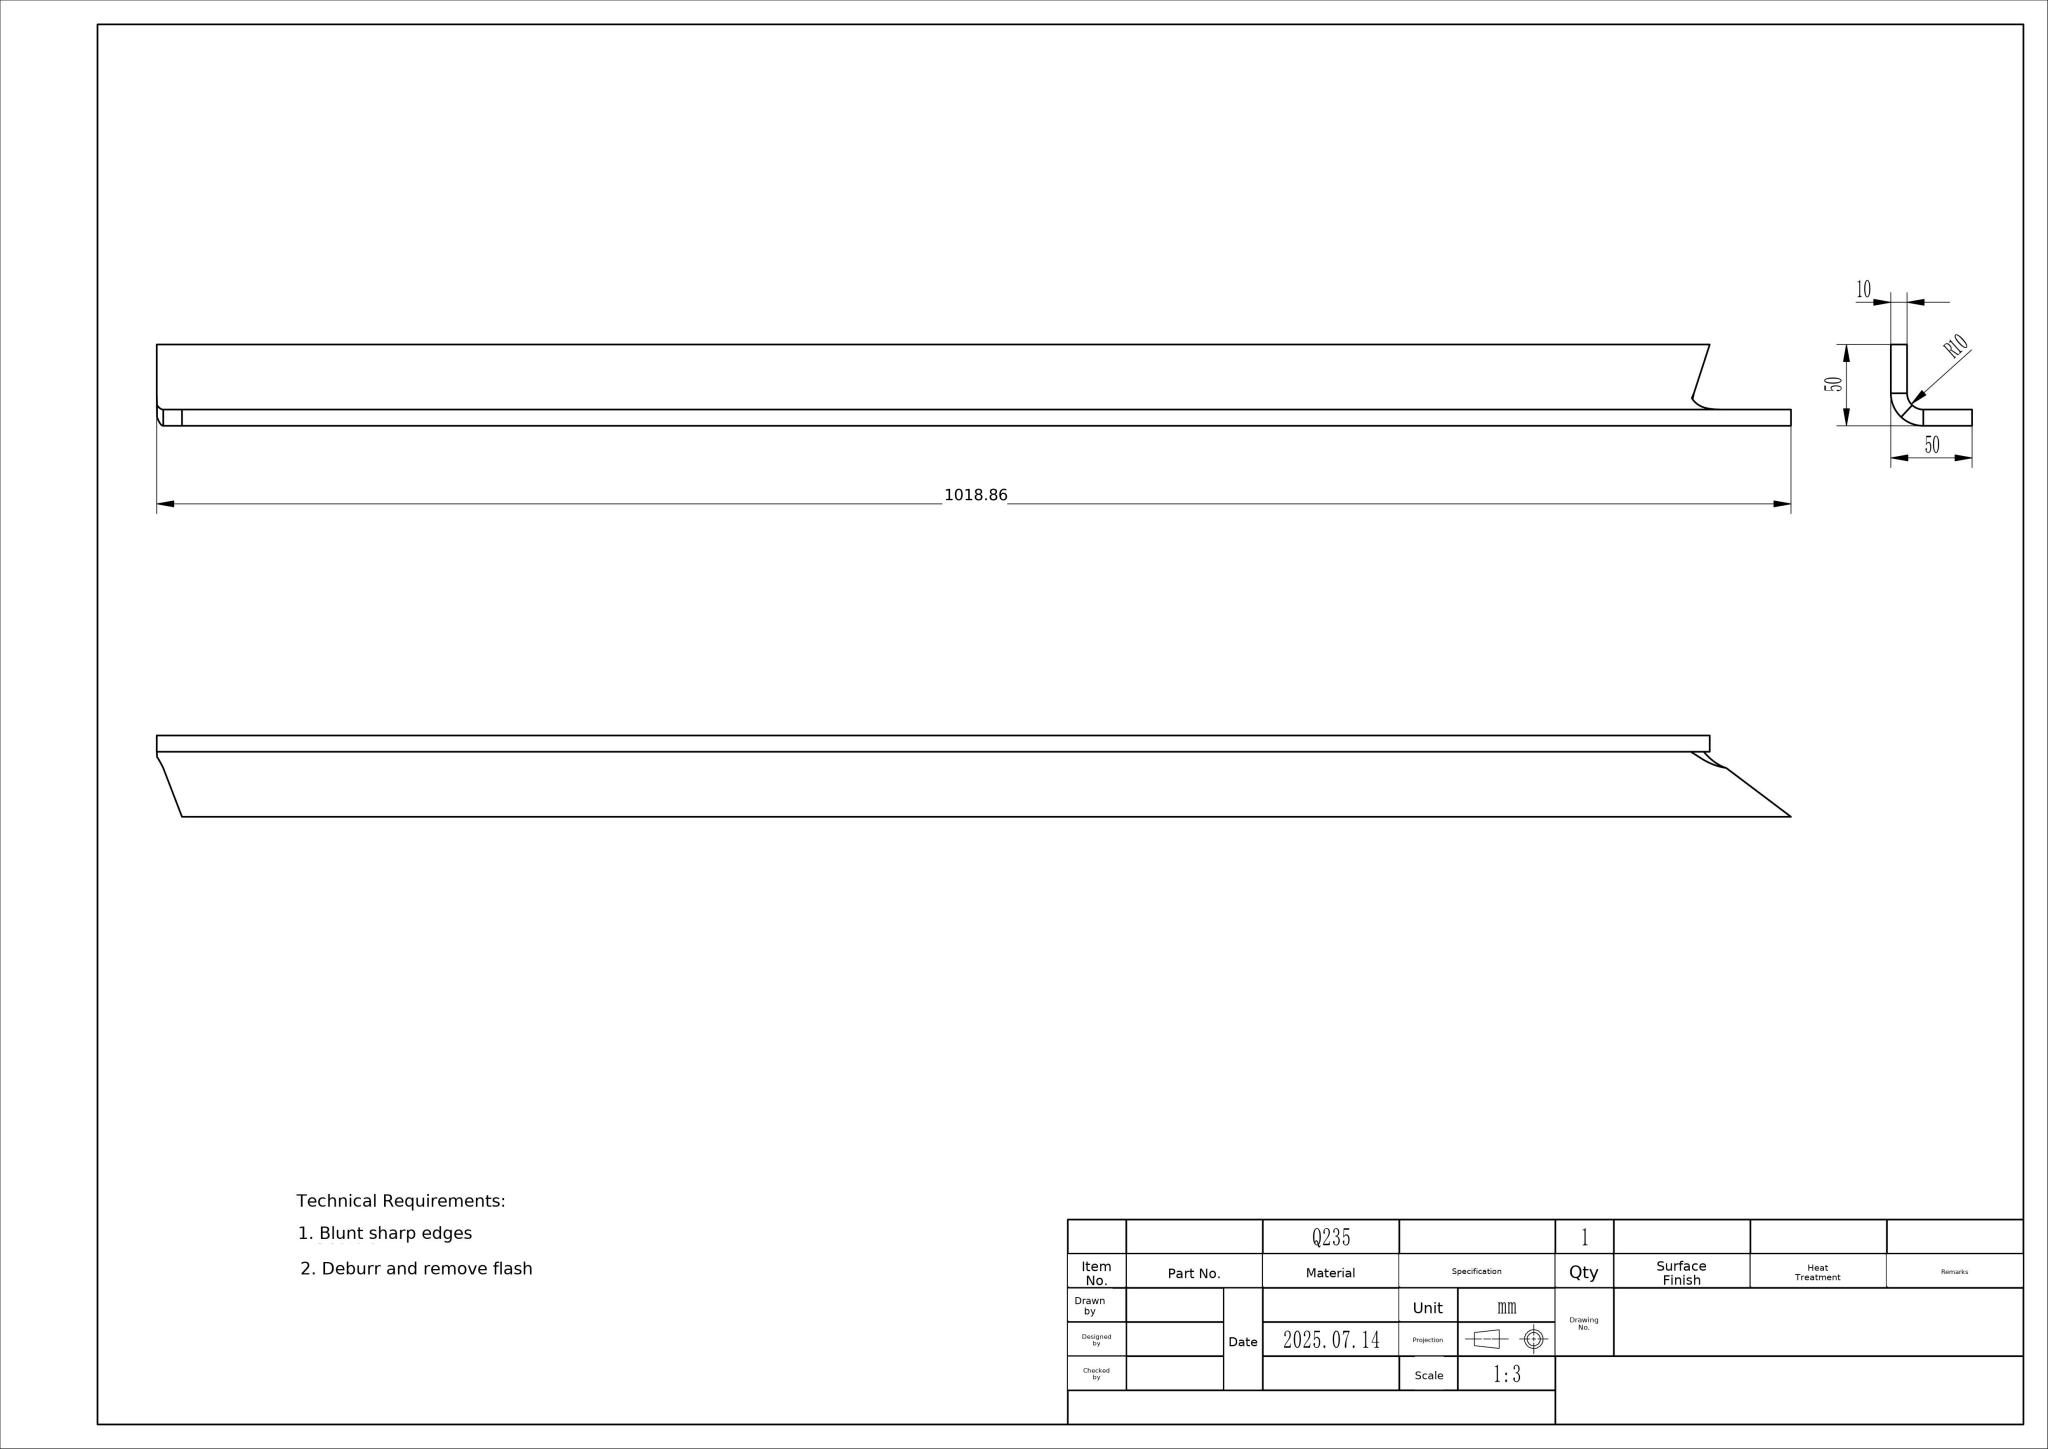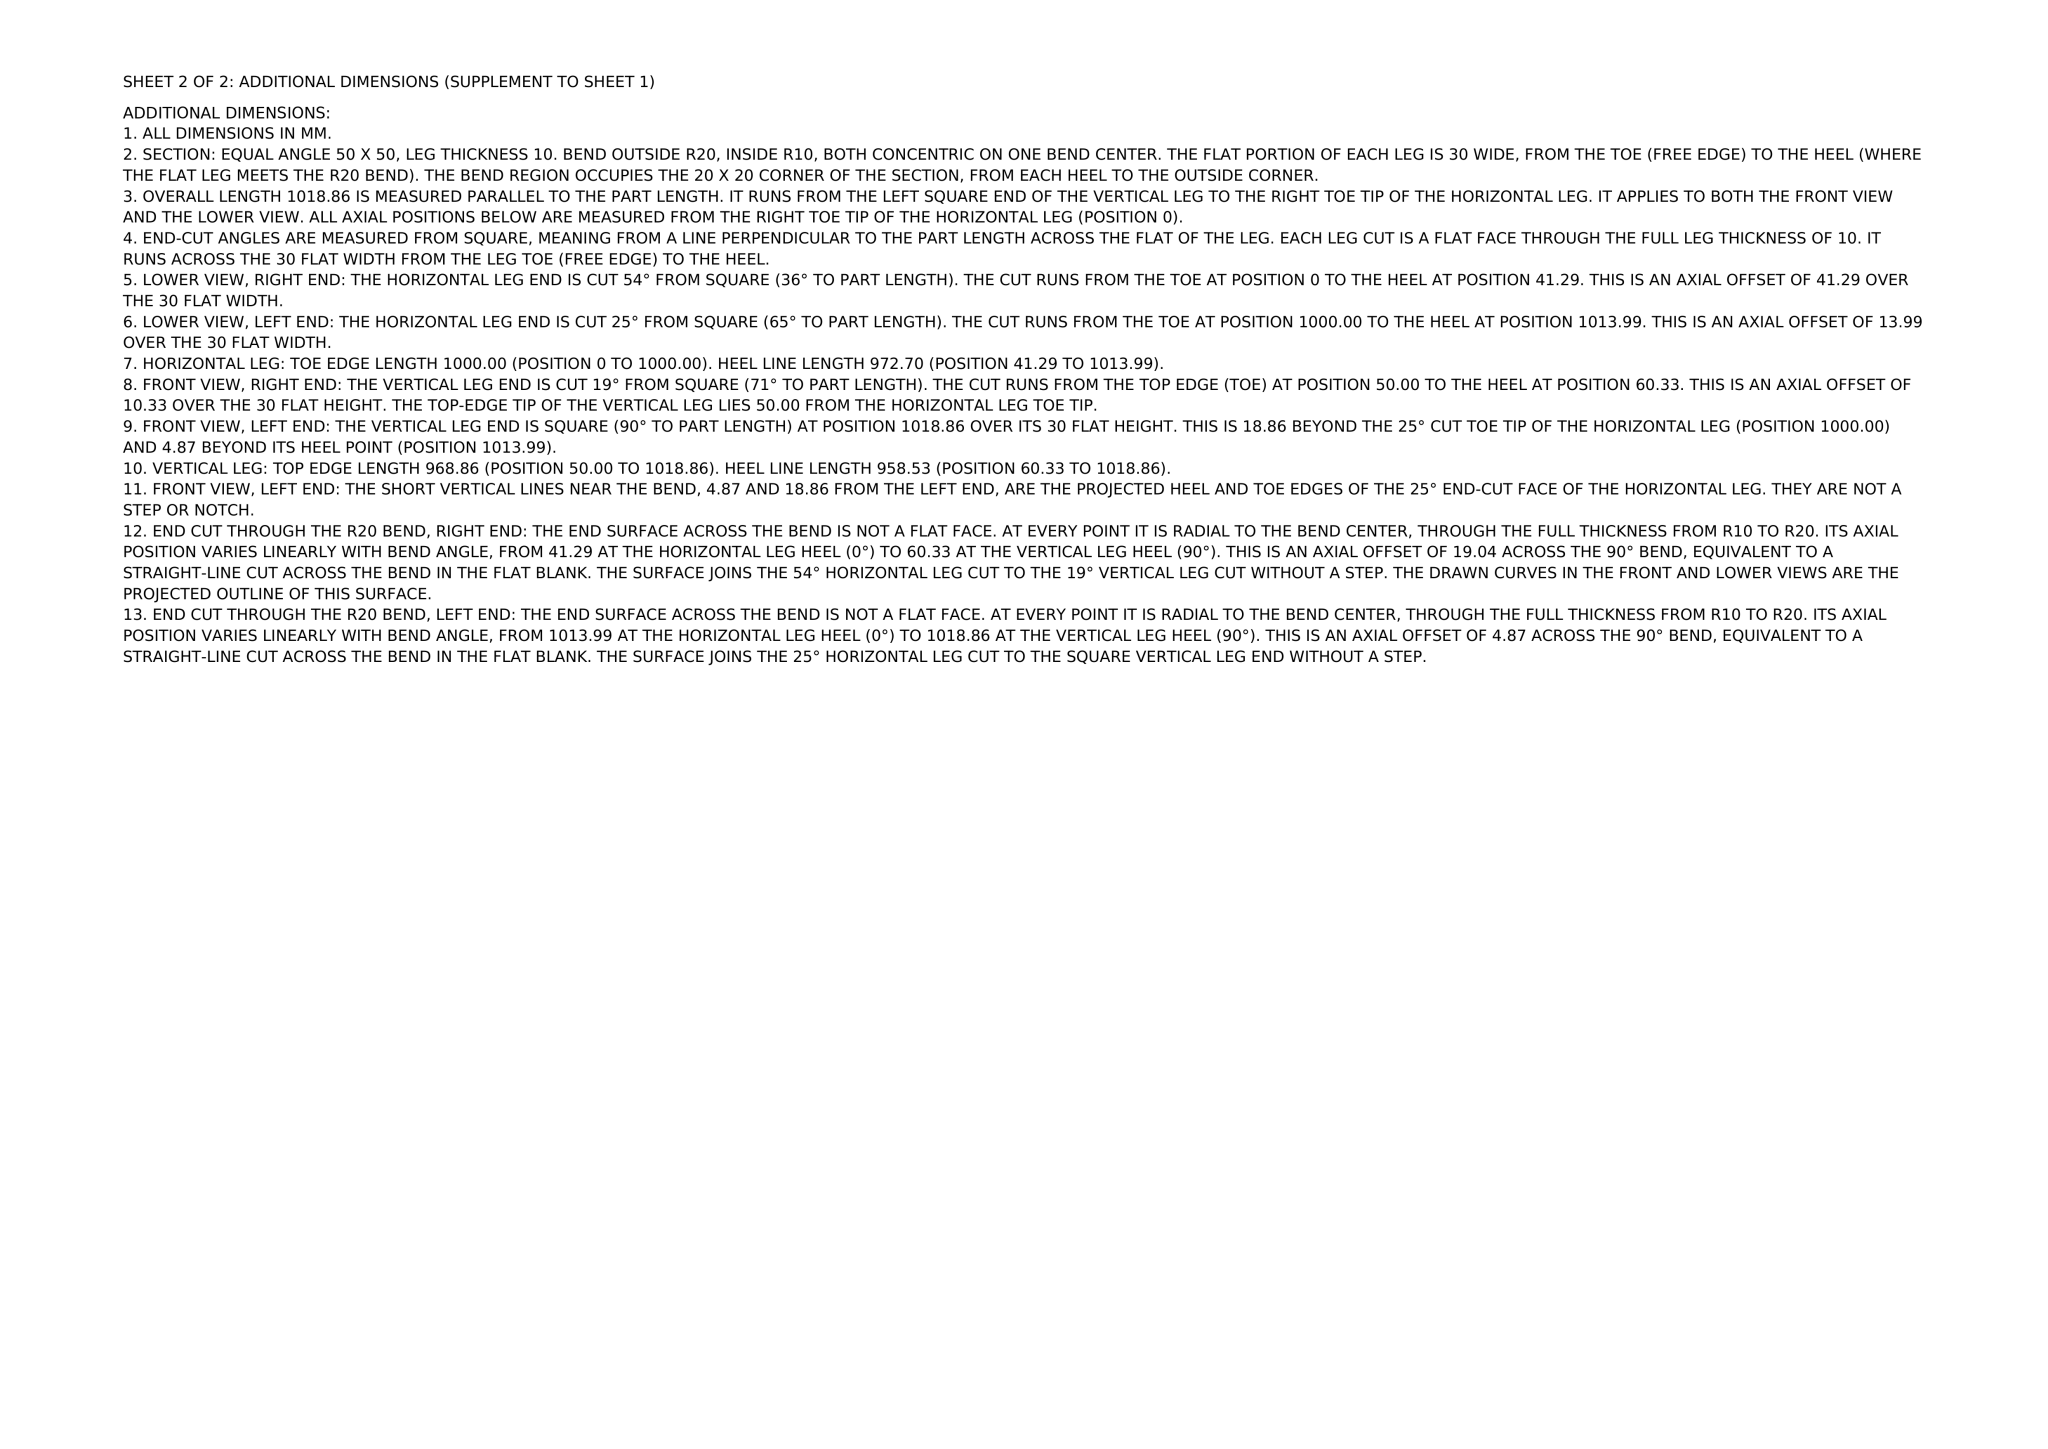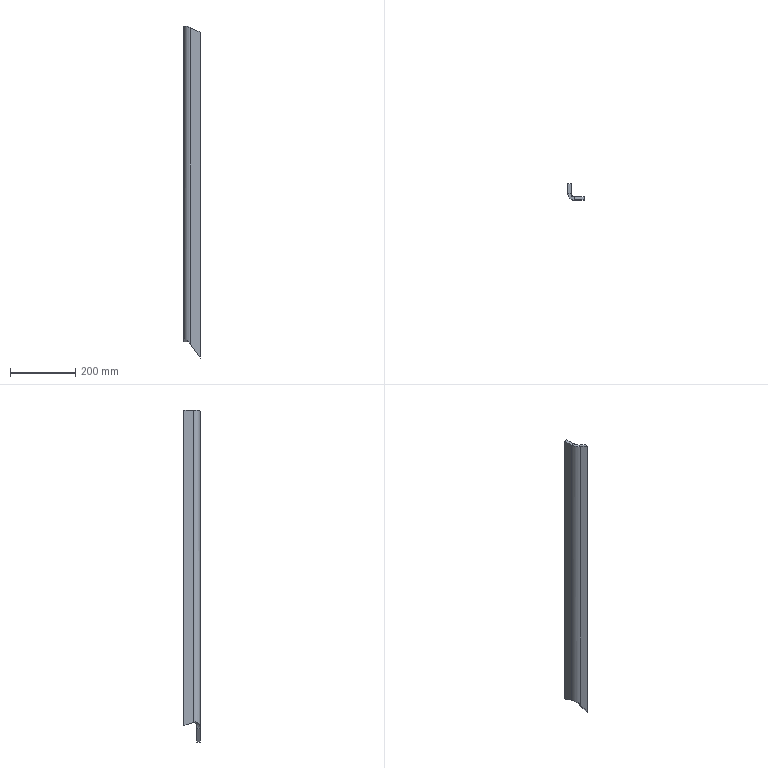Part | NX | mm | 1 solid | 16 faces | box 50 x 50 x 1018.86 mm | volume 811592 mm3 | plane 10 | spline 4 | cylinder 2 | commonest cylinder face diameters 40 x1 20 x1
STEP:
#1=CARTESIAN_POINT('',(0.,0.,0.));
#2=DIRECTION('',(0.,0.,1.));
#3=DIRECTION('',(1.,0.,0.));
#4=AXIS2_PLACEMENT_3D('',#1,#2,#3);
#5=(LENGTH_UNIT()NAMED_UNIT(*)SI_UNIT(.MILLI.,.METRE.));
#6=UNCERTAINTY_MEASURE_WITH_UNIT(LENGTH_MEASURE(0.0508),#5,'','');
#7=(NAMED_UNIT(*)PLANE_ANGLE_UNIT()SI_UNIT($,.RADIAN.));
#8=PLANE_ANGLE_MEASURE_WITH_UNIT(PLANE_ANGLE_MEASURE(0.01745),#7);
#9=DIMENSIONAL_EXPONENTS(0.,0.,0.,0.,0.,0.,0.);
#10=(CONVERSION_BASED_UNIT('',#8)NAMED_UNIT(#9)PLANE_ANGLE_UNIT());
#11=(NAMED_UNIT(*)SI_UNIT($,.STERADIAN.)SOLID_ANGLE_UNIT());
#12=(GEOMETRIC_REPRESENTATION_CONTEXT(3)GLOBAL_UNCERTAINTY_ASSIGNED_CONTEXT((#6))GLOBAL_UNIT_ASSIGNED_CONTEXT((#5,#10,#11))REPRESENTATION_CONTEXT('',''));
#13=SHAPE_REPRESENTATION('',(#4),#12);
#14=CARTESIAN_POINT('',(-40.,40.,50.));
#15=VERTEX_POINT('',#14);
#16=CARTESIAN_POINT('',(-40.,10.,60.33));
#17=VERTEX_POINT('',#16);
#18=CARTESIAN_POINT('',(-40.,10.,60.33));
#19=DIRECTION('',(-0.,-0.9455,0.3256));
#20=VECTOR('',#19,1.);
#21=LINE('',#18,#20);
#22=EDGE_CURVE('',#15,#17,#21,.T.);
#23=ORIENTED_EDGE('',*,*,#22,.T.);
#24=CARTESIAN_POINT('',(-50.,10.,60.33));
#25=VERTEX_POINT('',#24);
#26=CARTESIAN_POINT('',(-50.,10.,60.33));
#27=DIRECTION('',(-1.,-0.,0.));
#28=VECTOR('',#27,1.);
#29=LINE('',#26,#28);
#30=EDGE_CURVE('',#17,#25,#29,.T.);
#31=ORIENTED_EDGE('',*,*,#30,.T.);
#32=CARTESIAN_POINT('',(-50.,40.,50.));
#33=VERTEX_POINT('',#32);
#34=CARTESIAN_POINT('',(-50.,19.631,57.013));
#35=DIRECTION('',(-0.,-0.9455,0.3256));
#36=VECTOR('',#35,1.);
#37=LINE('',#34,#36);
#38=EDGE_CURVE('',#33,#25,#37,.T.);
#39=ORIENTED_EDGE('',*,*,#38,.F.);
#40=CARTESIAN_POINT('',(-60.,40.,50.));
#41=DIRECTION('',(1.,-0.,-0.));
#42=VECTOR('',#41,1.);
#43=LINE('',#40,#42);
#44=EDGE_CURVE('',#33,#15,#43,.T.);
#45=ORIENTED_EDGE('',*,*,#44,.T.);
#46=EDGE_LOOP('',(#23,#31,#39,#45));
#47=FACE_OUTER_BOUND('',#46,.T.);
#48=CARTESIAN_POINT('',(-60.,10.,60.33));
#49=DIRECTION('',(0.,0.3256,0.9455));
#50=DIRECTION('',(-0.,-0.9455,0.3256));
#51=AXIS2_PLACEMENT_3D('',#48,#49,#50);
#52=PLANE('',#51);
#53=ADVANCED_FACE('',(#47),#52,.F.);
#54=CARTESIAN_POINT('',(-50.,40.,1018.86));
#55=VERTEX_POINT('',#54);
#56=CARTESIAN_POINT('',(-50.,10.,1018.86));
#57=VERTEX_POINT('',#56);
#58=CARTESIAN_POINT('',(-50.,40.,1018.86));
#59=DIRECTION('',(-0.,-1.,-0.));
#60=VECTOR('',#59,1.);
#61=LINE('',#58,#60);
#62=EDGE_CURVE('',#55,#57,#61,.T.);
#63=ORIENTED_EDGE('',*,*,#62,.T.);
#64=CARTESIAN_POINT('',(-40.,10.,1018.86));
#65=VERTEX_POINT('',#64);
#66=CARTESIAN_POINT('',(-40.,10.,1018.86));
#67=DIRECTION('',(-1.,0.,0.));
#68=VECTOR('',#67,1.);
#69=LINE('',#66,#68);
#70=EDGE_CURVE('',#65,#57,#69,.T.);
#71=ORIENTED_EDGE('',*,*,#70,.F.);
#72=CARTESIAN_POINT('',(-40.,40.,1018.86));
#73=VERTEX_POINT('',#72);
#74=CARTESIAN_POINT('',(-40.,40.,1018.86));
#75=DIRECTION('',(-0.,-1.,-0.));
#76=VECTOR('',#75,1.);
#77=LINE('',#74,#76);
#78=EDGE_CURVE('',#73,#65,#77,.T.);
#79=ORIENTED_EDGE('',*,*,#78,.F.);
#80=CARTESIAN_POINT('',(-50.,40.,1018.86));
#81=DIRECTION('',(1.,-0.,-0.));
#82=VECTOR('',#81,1.);
#83=LINE('',#80,#82);
#84=EDGE_CURVE('',#55,#73,#83,.T.);
#85=ORIENTED_EDGE('',*,*,#84,.F.);
#86=EDGE_LOOP('',(#63,#71,#79,#85));
#87=FACE_OUTER_BOUND('',#86,.T.);
#88=CARTESIAN_POINT('',(-50.,40.,1018.86));
#89=DIRECTION('',(0.,-0.,1.));
#90=DIRECTION('',(1.,0.,-0.));
#91=AXIS2_PLACEMENT_3D('',#88,#89,#90);
#92=PLANE('',#91);
#93=ADVANCED_FACE('',(#87),#92,.T.);
#94=CARTESIAN_POINT('',(-50.,40.,0.));
#95=DIRECTION('',(0.,0.,1.));
#96=VECTOR('',#95,1.);
#97=LINE('',#94,#96);
#98=EDGE_CURVE('',#33,#55,#97,.T.);
#99=ORIENTED_EDGE('',*,*,#98,.F.);
#100=ORIENTED_EDGE('',*,*,#38,.T.);
#101=CARTESIAN_POINT('',(-50.,10.,0.));
#102=DIRECTION('',(0.,0.,1.));
#103=VECTOR('',#102,1.);
#104=LINE('',#101,#103);
#105=EDGE_CURVE('',#25,#57,#104,.T.);
#106=ORIENTED_EDGE('',*,*,#105,.T.);
#107=ORIENTED_EDGE('',*,*,#62,.F.);
#108=EDGE_LOOP('',(#99,#100,#106,#107));
#109=FACE_OUTER_BOUND('',#108,.T.);
#110=CARTESIAN_POINT('',(-50.,0.,0.));
#111=DIRECTION('',(1.,-0.,-0.));
#112=DIRECTION('',(0.,1.,0.));
#113=AXIS2_PLACEMENT_3D('',#110,#111,#112);
#114=PLANE('',#113);
#115=ADVANCED_FACE('',(#109),#114,.F.);
#116=ORIENTED_EDGE('',*,*,#22,.F.);
#117=CARTESIAN_POINT('',(-40.,40.,0.));
#118=DIRECTION('',(0.,0.,1.));
#119=VECTOR('',#118,1.);
#120=LINE('',#117,#119);
#121=EDGE_CURVE('',#15,#73,#120,.T.);
#122=ORIENTED_EDGE('',*,*,#121,.T.);
#123=ORIENTED_EDGE('',*,*,#78,.T.);
#124=CARTESIAN_POINT('',(-40.,10.,-0.));
#125=DIRECTION('',(0.,0.,1.));
#126=VECTOR('',#125,1.);
#127=LINE('',#124,#126);
#128=EDGE_CURVE('',#17,#65,#127,.T.);
#129=ORIENTED_EDGE('',*,*,#128,.F.);
#130=EDGE_LOOP('',(#116,#122,#123,#129));
#131=FACE_OUTER_BOUND('',#130,.T.);
#132=CARTESIAN_POINT('',(-40.,0.,0.));
#133=DIRECTION('',(1.,-0.,-0.));
#134=DIRECTION('',(0.,1.,0.));
#135=AXIS2_PLACEMENT_3D('',#132,#133,#134);
#136=PLANE('',#135);
#137=ADVANCED_FACE('',(#131),#136,.T.);
#138=ORIENTED_EDGE('',*,*,#44,.F.);
#139=ORIENTED_EDGE('',*,*,#98,.T.);
#140=ORIENTED_EDGE('',*,*,#84,.T.);
#141=ORIENTED_EDGE('',*,*,#121,.F.);
#142=EDGE_LOOP('',(#138,#139,#140,#141));
#143=FACE_OUTER_BOUND('',#142,.T.);
#144=CARTESIAN_POINT('',(-50.,40.,0.));
#145=DIRECTION('',(0.,1.,-0.));
#146=DIRECTION('',(-1.,0.,0.));
#147=AXIS2_PLACEMENT_3D('',#144,#145,#146);
#148=PLANE('',#147);
#149=ADVANCED_FACE('',(#143),#148,.T.);
#150=CARTESIAN_POINT('',(-39.551,7.038,61.707));
#151=VERTEX_POINT('',#150);
#152=CARTESIAN_POINT('',(-49.102,4.075,61.707));
#153=VERTEX_POINT('',#152);
#154=CARTESIAN_POINT('',(-44.327,5.556,61.707));
#155=DIRECTION('',(-0.9551,-0.2962,0.));
#156=VECTOR('',#155,1.);
#157=LINE('',#154,#156);
#158=EDGE_CURVE('',#151,#153,#157,.T.);
#159=ORIENTED_EDGE('',*,*,#158,.F.);
#160=CARTESIAN_POINT('',(-30.,-0.,41.291));
#161=VERTEX_POINT('',#160);
#162=CARTESIAN_POINT('',(-39.551,7.038,61.707));
#163=CARTESIAN_POINT('',(-39.319,6.288,61.238));
#164=CARTESIAN_POINT('',(-39.004,5.587,60.71));
#165=CARTESIAN_POINT('',(-38.257,4.311,59.541));
#166=CARTESIAN_POINT('',(-37.826,3.737,58.901));
#167=CARTESIAN_POINT('',(-36.9,2.73,57.515));
#168=CARTESIAN_POINT('',(-36.406,2.297,56.77));
#169=CARTESIAN_POINT('',(-35.406,1.564,55.186));
#170=CARTESIAN_POINT('',(-34.899,1.265,54.346));
#171=CARTESIAN_POINT('',(-33.915,0.7818,52.584));
#172=CARTESIAN_POINT('',(-33.438,0.5977,51.661));
#173=CARTESIAN_POINT('',(-32.543,0.3173,49.744));
#174=CARTESIAN_POINT('',(-32.125,0.2208,48.75));
#175=CARTESIAN_POINT('',(-31.369,0.08678,46.704));
#176=CARTESIAN_POINT('',(-31.032,0.04903,45.651));
#177=CARTESIAN_POINT('',(-30.447,0.00567,43.501));
#178=CARTESIAN_POINT('',(-30.199,-0.,42.404));
#179=CARTESIAN_POINT('',(-30.,-0.,41.291));
#180=B_SPLINE_CURVE_WITH_KNOTS('',3,(#162,#163,#164,#165,#166,#167,#168,#169,#170,#171,#172,#173,#174,#175,#176,#177,#178,#179),.UNSPECIFIED.,.F.,.F.,(4,2,2,2,2,2,2,2,4),(0.,0.125,0.25,0.375,0.5,0.625,0.75,0.875,1.),.UNSPECIFIED.);
#181=EDGE_CURVE('',#151,#161,#180,.T.);
#182=ORIENTED_EDGE('',*,*,#181,.T.);
#183=CARTESIAN_POINT('',(-30.,-10.,41.291));
#184=VERTEX_POINT('',#183);
#185=CARTESIAN_POINT('',(-30.,-20.,41.291));
#186=DIRECTION('',(0.,-1.,0.));
#187=VECTOR('',#186,1.);
#188=LINE('',#185,#187);
#189=EDGE_CURVE('',#161,#184,#188,.T.);
#190=ORIENTED_EDGE('',*,*,#189,.T.);
#191=CARTESIAN_POINT('',(-30.,-10.,41.291));
#192=CARTESIAN_POINT('',(-30.398,-10.,42.404));
#193=CARTESIAN_POINT('',(-30.893,-9.989,43.501));
#194=CARTESIAN_POINT('',(-32.063,-9.902,45.651));
#195=CARTESIAN_POINT('',(-32.739,-9.826,46.704));
#196=CARTESIAN_POINT('',(-34.25,-9.558,48.75));
#197=CARTESIAN_POINT('',(-35.085,-9.365,49.744));
#198=CARTESIAN_POINT('',(-36.875,-8.805,51.661));
#199=CARTESIAN_POINT('',(-37.83,-8.436,52.584));
#200=CARTESIAN_POINT('',(-39.798,-7.47,54.346));
#201=CARTESIAN_POINT('',(-40.811,-6.872,55.186));
#202=CARTESIAN_POINT('',(-42.813,-5.407,56.77));
#203=CARTESIAN_POINT('',(-43.801,-4.54,57.515));
#204=CARTESIAN_POINT('',(-45.652,-2.525,58.901));
#205=CARTESIAN_POINT('',(-46.515,-1.377,59.541));
#206=CARTESIAN_POINT('',(-48.008,1.174,60.71));
#207=CARTESIAN_POINT('',(-48.637,2.577,61.238));
#208=CARTESIAN_POINT('',(-49.102,4.075,61.707));
#209=B_SPLINE_CURVE_WITH_KNOTS('',3,(#191,#192,#193,#194,#195,#196,#197,#198,#199,#200,#201,#202,#203,#204,#205,#206,#207,#208),.UNSPECIFIED.,.F.,.F.,(4,2,2,2,2,2,2,2,4),(0.,0.125,0.25,0.375,0.5,0.625,0.75,0.875,1.),.UNSPECIFIED.);
#210=EDGE_CURVE('',#184,#153,#209,.T.);
#211=ORIENTED_EDGE('',*,*,#210,.T.);
#212=EDGE_LOOP('',(#159,#182,#190,#211));
#213=FACE_OUTER_BOUND('',#212,.T.);
#214=CARTESIAN_POINT('',(-30.,-10.,41.291));
#215=CARTESIAN_POINT('',(-30.398,-10.,42.404));
#216=CARTESIAN_POINT('',(-30.893,-9.989,43.501));
#217=CARTESIAN_POINT('',(-32.063,-9.902,45.651));
#218=CARTESIAN_POINT('',(-32.739,-9.826,46.704));
#219=CARTESIAN_POINT('',(-34.25,-9.558,48.75));
#220=CARTESIAN_POINT('',(-35.085,-9.365,49.744));
#221=CARTESIAN_POINT('',(-36.875,-8.805,51.661));
#222=CARTESIAN_POINT('',(-37.83,-8.436,52.584));
#223=CARTESIAN_POINT('',(-39.798,-7.47,54.346));
#224=CARTESIAN_POINT('',(-40.811,-6.872,55.186));
#225=CARTESIAN_POINT('',(-42.813,-5.407,56.77));
#226=CARTESIAN_POINT('',(-43.801,-4.54,57.515));
#227=CARTESIAN_POINT('',(-45.652,-2.525,58.901));
#228=CARTESIAN_POINT('',(-46.515,-1.377,59.541));
#229=CARTESIAN_POINT('',(-48.008,1.174,60.71));
#230=CARTESIAN_POINT('',(-48.637,2.577,61.238));
#231=CARTESIAN_POINT('',(-49.102,4.075,61.707));
#232=CARTESIAN_POINT('',(-30.,-0.,41.291));
#233=CARTESIAN_POINT('',(-30.199,-0.,42.404));
#234=CARTESIAN_POINT('',(-30.447,0.00567,43.501));
#235=CARTESIAN_POINT('',(-31.032,0.04903,45.651));
#236=CARTESIAN_POINT('',(-31.369,0.08678,46.704));
#237=CARTESIAN_POINT('',(-32.125,0.2208,48.75));
#238=CARTESIAN_POINT('',(-32.543,0.3173,49.744));
#239=CARTESIAN_POINT('',(-33.438,0.5977,51.661));
#240=CARTESIAN_POINT('',(-33.915,0.7818,52.584));
#241=CARTESIAN_POINT('',(-34.899,1.265,54.346));
#242=CARTESIAN_POINT('',(-35.406,1.564,55.186));
#243=CARTESIAN_POINT('',(-36.406,2.297,56.77));
#244=CARTESIAN_POINT('',(-36.9,2.73,57.515));
#245=CARTESIAN_POINT('',(-37.826,3.737,58.901));
#246=CARTESIAN_POINT('',(-38.257,4.311,59.541));
#247=CARTESIAN_POINT('',(-39.004,5.587,60.71));
#248=CARTESIAN_POINT('',(-39.319,6.288,61.238));
#249=CARTESIAN_POINT('',(-39.551,7.038,61.707));
#250=B_SPLINE_SURFACE_WITH_KNOTS('',1,3,((#214,#215,#216,#217,#218,#219,#220,#221,#222,#223,#224,#225,#226,#227,#228,#229,#230,#231),(#232,#233,#234,#235,#236,#237,#238,#239,#240,#241,#242,#243,#244,#245,#246,#247,#248,#249)),.UNSPECIFIED.,.F.,.F.,.F.,(2,2),(4,2,2,2,2,2,2,2,4),(0.,1.),(0.,0.125,0.25,0.375,0.5,0.625,0.75,0.875,1.),.UNSPECIFIED.);
#251=ADVANCED_FACE('',(#213),#250,.F.);
#252=CARTESIAN_POINT('',(-30.,-0.,1013.989));
#253=VERTEX_POINT('',#252);
#254=CARTESIAN_POINT('',(-30.,-10.,1013.989));
#255=VERTEX_POINT('',#254);
#256=CARTESIAN_POINT('',(-30.,-10.,1013.989));
#257=DIRECTION('',(0.,-1.,0.));
#258=VECTOR('',#257,1.);
#259=LINE('',#256,#258);
#260=EDGE_CURVE('',#253,#255,#259,.T.);
#261=ORIENTED_EDGE('',*,*,#260,.F.);
#262=CARTESIAN_POINT('',(-36.83,2.696,1018.652));
#263=VERTEX_POINT('',#262);
#264=CARTESIAN_POINT('',(-30.,-0.,1013.989));
#265=CARTESIAN_POINT('',(-30.627,-0.,1014.378));
#266=CARTESIAN_POINT('',(-31.253,0.05907,1014.766));
#267=CARTESIAN_POINT('',(-32.484,0.2932,1015.544));
#268=CARTESIAN_POINT('',(-33.089,0.4683,1015.932));
#269=CARTESIAN_POINT('',(-34.254,0.9284,1016.709));
#270=CARTESIAN_POINT('',(-34.815,1.213,1017.098));
#271=CARTESIAN_POINT('',(-35.875,1.883,1017.875));
#272=CARTESIAN_POINT('',(-36.372,2.268,1018.264));
#273=CARTESIAN_POINT('',(-36.83,2.696,1018.652));
#274=B_SPLINE_CURVE_WITH_KNOTS('',3,(#264,#265,#266,#267,#268,#269,#270,#271,#272,#273),.UNSPECIFIED.,.F.,.F.,(4,2,2,2,4),(0.,0.25,0.5,0.75,1.),.UNSPECIFIED.);
#275=EDGE_CURVE('',#253,#263,#274,.T.);
#276=ORIENTED_EDGE('',*,*,#275,.T.);
#277=CARTESIAN_POINT('',(-43.66,-4.608,1018.652));
#278=VERTEX_POINT('',#277);
#279=CARTESIAN_POINT('',(-36.83,2.696,1018.652));
#280=CARTESIAN_POINT('',(-37.4,2.086,1018.652));
#281=CARTESIAN_POINT('',(-37.971,1.476,1018.652));
#282=CARTESIAN_POINT('',(-38.541,0.8663,1018.652));
#283=CARTESIAN_POINT('',(-39.111,0.2565,1018.652));
#284=CARTESIAN_POINT('',(-39.682,-0.3534,1018.652));
#285=CARTESIAN_POINT('',(-40.252,-0.9633,1018.652));
#286=CARTESIAN_POINT('',(-41.388,-2.178,1018.652));
#287=CARTESIAN_POINT('',(-42.524,-3.393,1018.652));
#288=CARTESIAN_POINT('',(-43.66,-4.608,1018.652));
#289=B_SPLINE_CURVE_WITH_KNOTS('',3,(#279,#280,#281,#282,#283,#284,#285,#286,#287,#288),.UNSPECIFIED.,.F.,.F.,(4,3,3,4),(0.,0.2505,0.501,1.),.UNSPECIFIED.);
#290=EDGE_CURVE('',#263,#278,#289,.T.);
#291=ORIENTED_EDGE('',*,*,#290,.T.);
#292=CARTESIAN_POINT('',(-30.,-10.,1013.989));
#293=CARTESIAN_POINT('',(-35.013,-10.,1015.544));
#294=CARTESIAN_POINT('',(-39.999,-8.032,1017.098));
#295=CARTESIAN_POINT('',(-43.66,-4.608,1018.652));
#296=B_SPLINE_CURVE_WITH_KNOTS('',3,(#292,#293,#294,#295),.UNSPECIFIED.,.F.,.F.,(4,4),(0.,1.),.UNSPECIFIED.);
#297=EDGE_CURVE('',#255,#278,#296,.T.);
#298=ORIENTED_EDGE('',*,*,#297,.F.);
#299=EDGE_LOOP('',(#261,#276,#291,#298));
#300=FACE_OUTER_BOUND('',#299,.T.);
#301=CARTESIAN_POINT('',(-30.,-10.1,1013.989));
#302=CARTESIAN_POINT('',(-31.259,-10.1,1014.378));
#303=CARTESIAN_POINT('',(-32.519,-9.981,1014.766));
#304=CARTESIAN_POINT('',(-34.993,-9.511,1015.544));
#305=CARTESIAN_POINT('',(-36.208,-9.159,1015.932));
#306=CARTESIAN_POINT('',(-38.551,-8.234,1016.709));
#307=CARTESIAN_POINT('',(-39.679,-7.661,1017.098));
#308=CARTESIAN_POINT('',(-41.808,-6.315,1017.875));
#309=CARTESIAN_POINT('',(-42.809,-5.541,1018.264));
#310=CARTESIAN_POINT('',(-43.729,-4.681,1018.652));
#311=CARTESIAN_POINT('',(-30.,-10.,1013.989));
#312=CARTESIAN_POINT('',(-31.253,-10.,1014.378));
#313=CARTESIAN_POINT('',(-32.506,-9.882,1014.766));
#314=CARTESIAN_POINT('',(-34.968,-9.414,1015.544));
#315=CARTESIAN_POINT('',(-36.177,-9.063,1015.932));
#316=CARTESIAN_POINT('',(-38.509,-8.143,1016.709));
#317=CARTESIAN_POINT('',(-39.631,-7.573,1017.098));
#318=CARTESIAN_POINT('',(-41.749,-6.234,1017.875));
#319=CARTESIAN_POINT('',(-42.745,-5.464,1018.264));
#320=CARTESIAN_POINT('',(-43.66,-4.608,1018.652));
#321=CARTESIAN_POINT('',(-30.,-0.,1013.989));
#322=CARTESIAN_POINT('',(-30.627,-0.,1014.378));
#323=CARTESIAN_POINT('',(-31.253,0.05907,1014.766));
#324=CARTESIAN_POINT('',(-32.484,0.2932,1015.544));
#325=CARTESIAN_POINT('',(-33.089,0.4683,1015.932));
#326=CARTESIAN_POINT('',(-34.254,0.9284,1016.709));
#327=CARTESIAN_POINT('',(-34.815,1.213,1017.098));
#328=CARTESIAN_POINT('',(-35.875,1.883,1017.875));
#329=CARTESIAN_POINT('',(-36.372,2.268,1018.264));
#330=CARTESIAN_POINT('',(-36.83,2.696,1018.652));
#331=B_SPLINE_SURFACE_WITH_KNOTS('',1,3,((#301,#302,#303,#304,#305,#306,#307,#308,#309,#310),(#311,#312,#313,#314,#315,#316,#317,#318,#319,#320),(#321,#322,#323,#324,#325,#326,#327,#328,#329,#330)),.UNSPECIFIED.,.F.,.F.,.F.,(2,1,2),(4,2,2,2,4),(0.,0.009901,1.),(0.,0.25,0.5,0.75,1.),.UNSPECIFIED.);
#332=ADVANCED_FACE('',(#300),#331,.T.);
#333=ORIENTED_EDGE('',*,*,#290,.F.);
#334=CARTESIAN_POINT('',(-36.83,2.696,1018.652));
#335=CARTESIAN_POINT('',(-37.329,3.162,1018.67));
#336=CARTESIAN_POINT('',(-37.779,3.679,1018.687));
#337=CARTESIAN_POINT('',(-38.566,4.795,1018.722));
#338=CARTESIAN_POINT('',(-38.902,5.393,1018.739));
#339=CARTESIAN_POINT('',(-39.445,6.645,1018.774));
#340=CARTESIAN_POINT('',(-39.652,7.299,1018.791));
#341=CARTESIAN_POINT('',(-39.93,8.635,1018.826));
#342=CARTESIAN_POINT('',(-40.,9.318,1018.843));
#343=CARTESIAN_POINT('',(-40.,10.,1018.86));
#344=B_SPLINE_CURVE_WITH_KNOTS('',3,(#334,#335,#336,#337,#338,#339,#340,#341,#342,#343),.UNSPECIFIED.,.F.,.F.,(4,2,2,2,4),(0.,0.25,0.5,0.75,1.),.UNSPECIFIED.);
#345=EDGE_CURVE('',#263,#65,#344,.T.);
#346=ORIENTED_EDGE('',*,*,#345,.T.);
#347=ORIENTED_EDGE('',*,*,#70,.T.);
#348=CARTESIAN_POINT('',(-43.66,-4.608,1018.652));
#349=CARTESIAN_POINT('',(-47.648,-0.8793,1018.722));
#350=CARTESIAN_POINT('',(-50.,4.541,1018.791));
#351=CARTESIAN_POINT('',(-50.,10.,1018.86));
#352=B_SPLINE_CURVE_WITH_KNOTS('',3,(#348,#349,#350,#351),.UNSPECIFIED.,.F.,.F.,(4,4),(0.,1.),.UNSPECIFIED.);
#353=EDGE_CURVE('',#278,#57,#352,.T.);
#354=ORIENTED_EDGE('',*,*,#353,.F.);
#355=EDGE_LOOP('',(#333,#346,#347,#354));
#356=FACE_OUTER_BOUND('',#355,.T.);
#357=CARTESIAN_POINT('',(-43.729,-4.681,1018.652));
#358=CARTESIAN_POINT('',(-44.73,-3.744,1018.67));
#359=CARTESIAN_POINT('',(-45.636,-2.705,1018.687));
#360=CARTESIAN_POINT('',(-47.217,-0.4625,1018.722));
#361=CARTESIAN_POINT('',(-47.892,0.7396,1018.739));
#362=CARTESIAN_POINT('',(-48.985,3.256,1018.774));
#363=CARTESIAN_POINT('',(-49.401,4.571,1018.791));
#364=CARTESIAN_POINT('',(-49.959,7.257,1018.826));
#365=CARTESIAN_POINT('',(-50.1,8.628,1018.843));
#366=CARTESIAN_POINT('',(-50.1,10.,1018.86));
#367=CARTESIAN_POINT('',(-43.66,-4.608,1018.652));
#368=CARTESIAN_POINT('',(-44.657,-3.676,1018.67));
#369=CARTESIAN_POINT('',(-45.558,-2.641,1018.687));
#370=CARTESIAN_POINT('',(-47.131,-0.4105,1018.722));
#371=CARTESIAN_POINT('',(-47.803,0.7857,1018.739));
#372=CARTESIAN_POINT('',(-48.89,3.29,1018.774));
#373=CARTESIAN_POINT('',(-49.305,4.598,1018.791));
#374=CARTESIAN_POINT('',(-49.86,7.27,1018.826));
#375=CARTESIAN_POINT('',(-50.,8.635,1018.843));
#376=CARTESIAN_POINT('',(-50.,10.,1018.86));
#377=CARTESIAN_POINT('',(-36.83,2.696,1018.652));
#378=CARTESIAN_POINT('',(-37.329,3.162,1018.67));
#379=CARTESIAN_POINT('',(-37.779,3.679,1018.687));
#380=CARTESIAN_POINT('',(-38.566,4.795,1018.722));
#381=CARTESIAN_POINT('',(-38.902,5.393,1018.739));
#382=CARTESIAN_POINT('',(-39.445,6.645,1018.774));
#383=CARTESIAN_POINT('',(-39.652,7.299,1018.791));
#384=CARTESIAN_POINT('',(-39.93,8.635,1018.826));
#385=CARTESIAN_POINT('',(-40.,9.318,1018.843));
#386=CARTESIAN_POINT('',(-40.,10.,1018.86));
#387=B_SPLINE_SURFACE_WITH_KNOTS('',1,3,((#357,#358,#359,#360,#361,#362,#363,#364,#365,#366),(#367,#368,#369,#370,#371,#372,#373,#374,#375,#376),(#377,#378,#379,#380,#381,#382,#383,#384,#385,#386)),.UNSPECIFIED.,.F.,.F.,.F.,(2,1,2),(4,2,2,2,4),(0.,0.009901,1.),(0.,0.25,0.5,0.75,1.),.UNSPECIFIED.);
#388=ADVANCED_FACE('',(#356),#387,.T.);
#389=CARTESIAN_POINT('',(-40.,10.,60.33));
#390=CARTESIAN_POINT('',(-40.,8.997,60.789));
#391=CARTESIAN_POINT('',(-39.848,7.995,61.248));
#392=CARTESIAN_POINT('',(-39.551,7.038,61.707));
#393=B_SPLINE_CURVE_WITH_KNOTS('',3,(#389,#390,#391,#392),.UNSPECIFIED.,.F.,.F.,(4,4),(0.,1.),.UNSPECIFIED.);
#394=EDGE_CURVE('',#17,#151,#393,.T.);
#395=ORIENTED_EDGE('',*,*,#394,.T.);
#396=ORIENTED_EDGE('',*,*,#158,.T.);
#397=CARTESIAN_POINT('',(-49.102,4.075,61.707));
#398=CARTESIAN_POINT('',(-49.696,5.991,61.248));
#399=CARTESIAN_POINT('',(-50.,7.995,60.789));
#400=CARTESIAN_POINT('',(-50.,10.,60.33));
#401=B_SPLINE_CURVE_WITH_KNOTS('',3,(#397,#398,#399,#400),.UNSPECIFIED.,.F.,.F.,(4,4),(0.,1.),.UNSPECIFIED.);
#402=EDGE_CURVE('',#153,#25,#401,.T.);
#403=ORIENTED_EDGE('',*,*,#402,.T.);
#404=ORIENTED_EDGE('',*,*,#30,.F.);
#405=EDGE_LOOP('',(#395,#396,#403,#404));
#406=FACE_OUTER_BOUND('',#405,.T.);
#407=CARTESIAN_POINT('',(-49.102,4.075,61.707));
#408=CARTESIAN_POINT('',(-49.696,5.991,61.248));
#409=CARTESIAN_POINT('',(-50.,7.995,60.789));
#410=CARTESIAN_POINT('',(-50.,10.,60.33));
#411=CARTESIAN_POINT('',(-39.551,7.038,61.707));
#412=CARTESIAN_POINT('',(-39.848,7.995,61.248));
#413=CARTESIAN_POINT('',(-40.,8.997,60.789));
#414=CARTESIAN_POINT('',(-40.,10.,60.33));
#415=B_SPLINE_SURFACE_WITH_KNOTS('',1,3,((#407,#408,#409,#410),(#411,#412,#413,#414)),.UNSPECIFIED.,.F.,.F.,.F.,(2,2),(4,4),(0.,1.),(0.,1.),.UNSPECIFIED.);
#416=ADVANCED_FACE('',(#406),#415,.F.);
#417=ORIENTED_EDGE('',*,*,#105,.F.);
#418=ORIENTED_EDGE('',*,*,#402,.F.);
#419=ORIENTED_EDGE('',*,*,#210,.F.);
#420=CARTESIAN_POINT('',(-30.,-10.,1013.989));
#421=DIRECTION('',(0.,0.,-1.));
#422=VECTOR('',#421,1.);
#423=LINE('',#420,#422);
#424=EDGE_CURVE('',#255,#184,#423,.T.);
#425=ORIENTED_EDGE('',*,*,#424,.F.);
#426=ORIENTED_EDGE('',*,*,#297,.T.);
#427=ORIENTED_EDGE('',*,*,#353,.T.);
#428=EDGE_LOOP('',(#417,#418,#419,#425,#426,#427));
#429=FACE_OUTER_BOUND('',#428,.T.);
#430=CARTESIAN_POINT('',(-30.,10.,1013.989));
#431=DIRECTION('',(-0.,-0.,-1.));
#432=DIRECTION('',(-0.,1.,0.));
#433=AXIS2_PLACEMENT_3D('',#430,#431,#432);
#434=CYLINDRICAL_SURFACE('',#433,20.);
#435=ADVANCED_FACE('',(#429),#434,.T.);
#436=ORIENTED_EDGE('',*,*,#128,.T.);
#437=ORIENTED_EDGE('',*,*,#345,.F.);
#438=ORIENTED_EDGE('',*,*,#275,.F.);
#439=CARTESIAN_POINT('',(-30.,-0.,1013.989));
#440=DIRECTION('',(0.,0.,-1.));
#441=VECTOR('',#440,1.);
#442=LINE('',#439,#441);
#443=EDGE_CURVE('',#253,#161,#442,.T.);
#444=ORIENTED_EDGE('',*,*,#443,.T.);
#445=ORIENTED_EDGE('',*,*,#181,.F.);
#446=ORIENTED_EDGE('',*,*,#394,.F.);
#447=EDGE_LOOP('',(#436,#437,#438,#444,#445,#446));
#448=FACE_OUTER_BOUND('',#447,.T.);
#449=CARTESIAN_POINT('',(-30.,10.,1013.989));
#450=DIRECTION('',(-0.,-0.,-1.));
#451=DIRECTION('',(-0.,1.,0.));
#452=AXIS2_PLACEMENT_3D('',#449,#450,#451);
#453=CYLINDRICAL_SURFACE('',#452,10.);
#454=ADVANCED_FACE('',(#448),#453,.F.);
#455=CARTESIAN_POINT('',(0.,0.,0.));
#456=VERTEX_POINT('',#455);
#457=CARTESIAN_POINT('',(-0.,0.,1000.));
#458=VERTEX_POINT('',#457);
#459=CARTESIAN_POINT('',(0.,0.,0.));
#460=DIRECTION('',(-0.,0.,1.));
#461=VECTOR('',#460,1.);
#462=LINE('',#459,#461);
#463=EDGE_CURVE('',#456,#458,#462,.T.);
#464=ORIENTED_EDGE('',*,*,#463,.T.);
#465=CARTESIAN_POINT('',(-0.,-10.,1000.));
#466=VERTEX_POINT('',#465);
#467=CARTESIAN_POINT('',(-0.,-10.,1000.));
#468=DIRECTION('',(0.,-1.,0.));
#469=VECTOR('',#468,1.);
#470=LINE('',#467,#469);
#471=EDGE_CURVE('',#458,#466,#470,.T.);
#472=ORIENTED_EDGE('',*,*,#471,.T.);
#473=CARTESIAN_POINT('',(0.,-10.,0.));
#474=VERTEX_POINT('',#473);
#475=CARTESIAN_POINT('',(0.,-10.,0.));
#476=DIRECTION('',(-0.,0.,1.));
#477=VECTOR('',#476,1.);
#478=LINE('',#475,#477);
#479=EDGE_CURVE('',#474,#466,#478,.T.);
#480=ORIENTED_EDGE('',*,*,#479,.F.);
#481=CARTESIAN_POINT('',(0.,-10.,0.));
#482=DIRECTION('',(0.,-1.,0.));
#483=VECTOR('',#482,1.);
#484=LINE('',#481,#483);
#485=EDGE_CURVE('',#456,#474,#484,.T.);
#486=ORIENTED_EDGE('',*,*,#485,.F.);
#487=EDGE_LOOP('',(#464,#472,#480,#486));
#488=FACE_OUTER_BOUND('',#487,.T.);
#489=CARTESIAN_POINT('',(0.,-10.,0.));
#490=DIRECTION('',(-1.,0.,-0.));
#491=DIRECTION('',(-0.,0.,1.));
#492=AXIS2_PLACEMENT_3D('',#489,#490,#491);
#493=PLANE('',#492);
#494=ADVANCED_FACE('',(#488),#493,.F.);
#495=CARTESIAN_POINT('',(-30.,0.,41.291));
#496=DIRECTION('',(0.5878,-0.,-0.809));
#497=VECTOR('',#496,1.);
#498=LINE('',#495,#497);
#499=EDGE_CURVE('',#161,#456,#498,.T.);
#500=ORIENTED_EDGE('',*,*,#499,.F.);
#501=ORIENTED_EDGE('',*,*,#443,.F.);
#502=CARTESIAN_POINT('',(-0.,0.,1000.));
#503=DIRECTION('',(-0.9063,-0.,0.4226));
#504=VECTOR('',#503,1.);
#505=LINE('',#502,#504);
#506=EDGE_CURVE('',#458,#253,#505,.T.);
#507=ORIENTED_EDGE('',*,*,#506,.F.);
#508=ORIENTED_EDGE('',*,*,#463,.F.);
#509=EDGE_LOOP('',(#500,#501,#507,#508));
#510=FACE_OUTER_BOUND('',#509,.T.);
#511=CARTESIAN_POINT('',(-0.,0.,-0.));
#512=DIRECTION('',(-0.,1.,-0.));
#513=DIRECTION('',(-1.,-0.,0.));
#514=AXIS2_PLACEMENT_3D('',#511,#512,#513);
#515=PLANE('',#514);
#516=ADVANCED_FACE('',(#510),#515,.T.);
#517=ORIENTED_EDGE('',*,*,#260,.T.);
#518=CARTESIAN_POINT('',(-0.,-10.,1000.));
#519=DIRECTION('',(-0.9063,-0.,0.4226));
#520=VECTOR('',#519,1.);
#521=LINE('',#518,#520);
#522=EDGE_CURVE('',#466,#255,#521,.T.);
#523=ORIENTED_EDGE('',*,*,#522,.F.);
#524=ORIENTED_EDGE('',*,*,#471,.F.);
#525=ORIENTED_EDGE('',*,*,#506,.T.);
#526=EDGE_LOOP('',(#517,#523,#524,#525));
#527=FACE_OUTER_BOUND('',#526,.T.);
#528=CARTESIAN_POINT('',(-0.,-10.,1000.));
#529=DIRECTION('',(-0.4226,0.,-0.9063));
#530=DIRECTION('',(-0.9063,0.,0.4226));
#531=AXIS2_PLACEMENT_3D('',#528,#529,#530);
#532=PLANE('',#531);
#533=ADVANCED_FACE('',(#527),#532,.F.);
#534=ORIENTED_EDGE('',*,*,#424,.T.);
#535=CARTESIAN_POINT('',(-0.,-10.,-0.));
#536=DIRECTION('',(0.5878,0.,-0.809));
#537=VECTOR('',#536,1.);
#538=LINE('',#535,#537);
#539=EDGE_CURVE('',#184,#474,#538,.T.);
#540=ORIENTED_EDGE('',*,*,#539,.T.);
#541=ORIENTED_EDGE('',*,*,#479,.T.);
#542=ORIENTED_EDGE('',*,*,#522,.T.);
#543=EDGE_LOOP('',(#534,#540,#541,#542));
#544=FACE_OUTER_BOUND('',#543,.T.);
#545=CARTESIAN_POINT('',(-0.,-10.,-0.));
#546=DIRECTION('',(-0.,1.,-0.));
#547=DIRECTION('',(-1.,-0.,0.));
#548=AXIS2_PLACEMENT_3D('',#545,#546,#547);
#549=PLANE('',#548);
#550=ADVANCED_FACE('',(#544),#549,.F.);
#551=ORIENTED_EDGE('',*,*,#189,.F.);
#552=ORIENTED_EDGE('',*,*,#499,.T.);
#553=ORIENTED_EDGE('',*,*,#485,.T.);
#554=ORIENTED_EDGE('',*,*,#539,.F.);
#555=EDGE_LOOP('',(#551,#552,#553,#554));
#556=FACE_OUTER_BOUND('',#555,.T.);
#557=CARTESIAN_POINT('',(-30.,-20.,41.291));
#558=DIRECTION('',(0.809,0.,0.5878));
#559=DIRECTION('',(0.5878,0.,-0.809));
#560=AXIS2_PLACEMENT_3D('',#557,#558,#559);
#561=PLANE('',#560);
#562=ADVANCED_FACE('',(#556),#561,.F.);
#563=CLOSED_SHELL('',(#53,#93,#115,#137,#149,#251,#332,#388,#416,#435,#454,#494,#516,#533,#550,#562));
#564=MANIFOLD_SOLID_BREP('',#563);
#565=ADVANCED_BREP_SHAPE_REPRESENTATION('',(#564),#12);
#566=SHAPE_REPRESENTATION_RELATIONSHIP('','',#13,#565);
#567=PRESENTATION_LAYER_ASSIGNMENT('','',(#564));
#568=COLOUR_RGB('',0.5961,0.6667,0.6863);
#569=FILL_AREA_STYLE_COLOUR('',#568);
#570=FILL_AREA_STYLE('',(#569));
#571=SURFACE_STYLE_FILL_AREA(#570);
#572=SURFACE_SIDE_STYLE('',(#571));
#573=SURFACE_STYLE_USAGE(.BOTH.,#572);
#574=PRESENTATION_STYLE_ASSIGNMENT((#573));
#575=STYLED_ITEM('',(#574),#564);
#576=MECHANICAL_DESIGN_GEOMETRIC_PRESENTATION_REPRESENTATION('',(#575),#12);